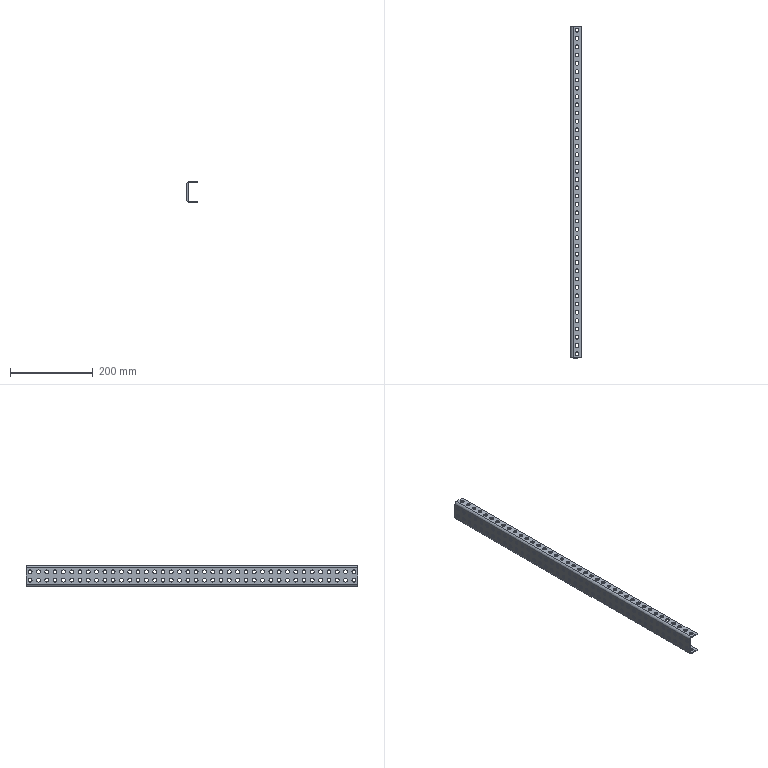Component | SolidWorks | MiddleColumnF2-1 | 1 solid | 342 faces | volume 186823 mm3 | cylinder 324 | plane 18 | commonest cylinder face diameters 9 x320 11 x2 5 x2